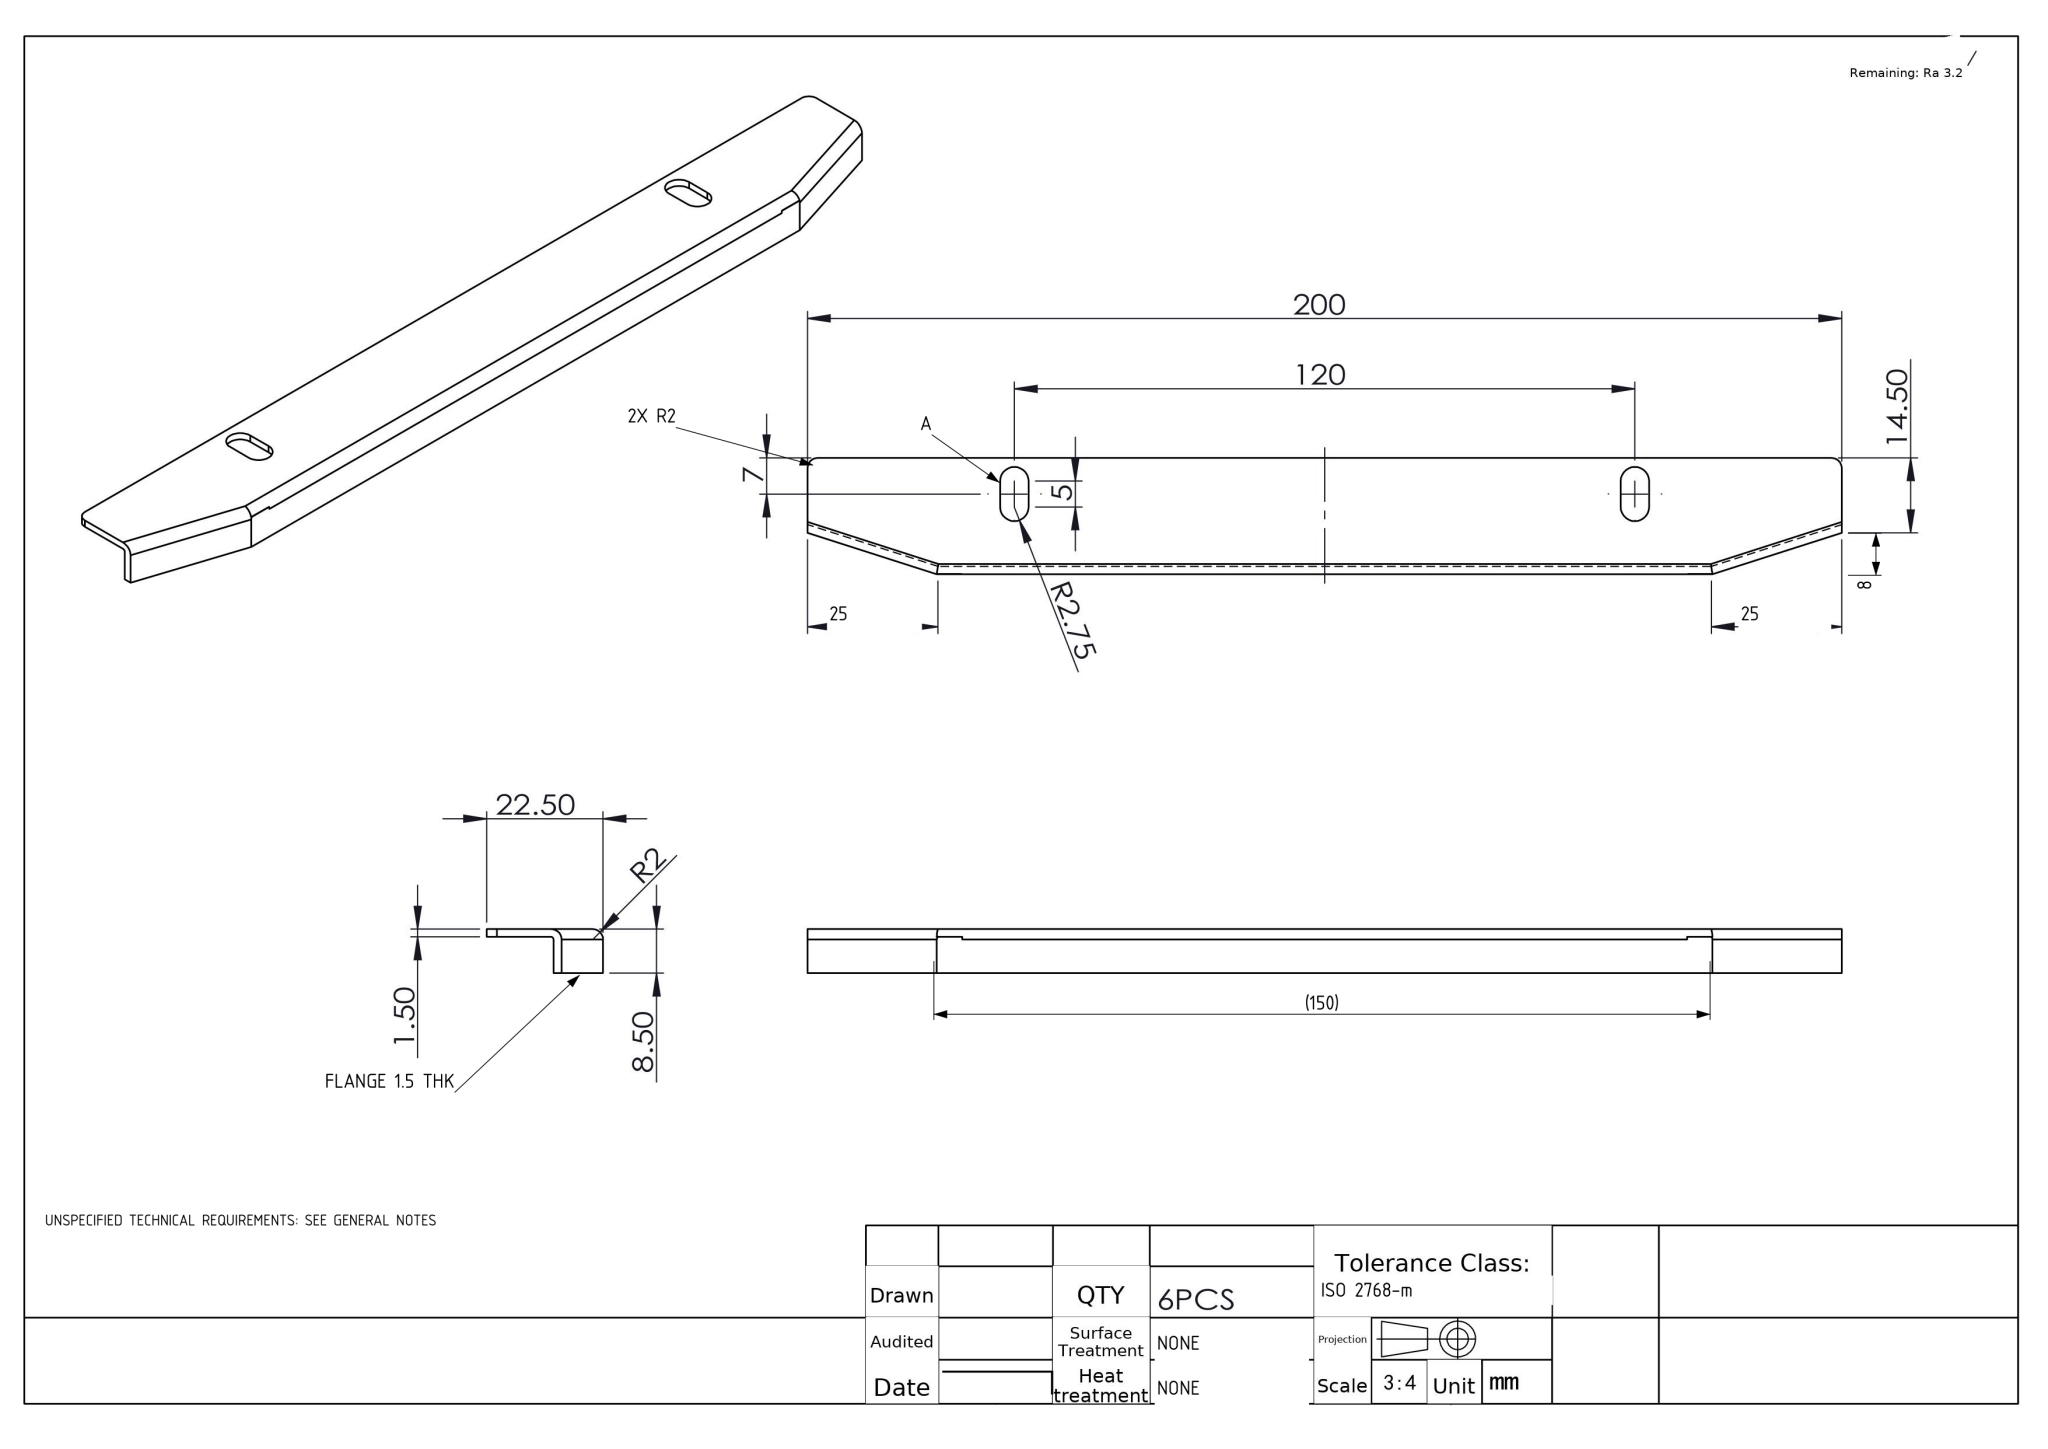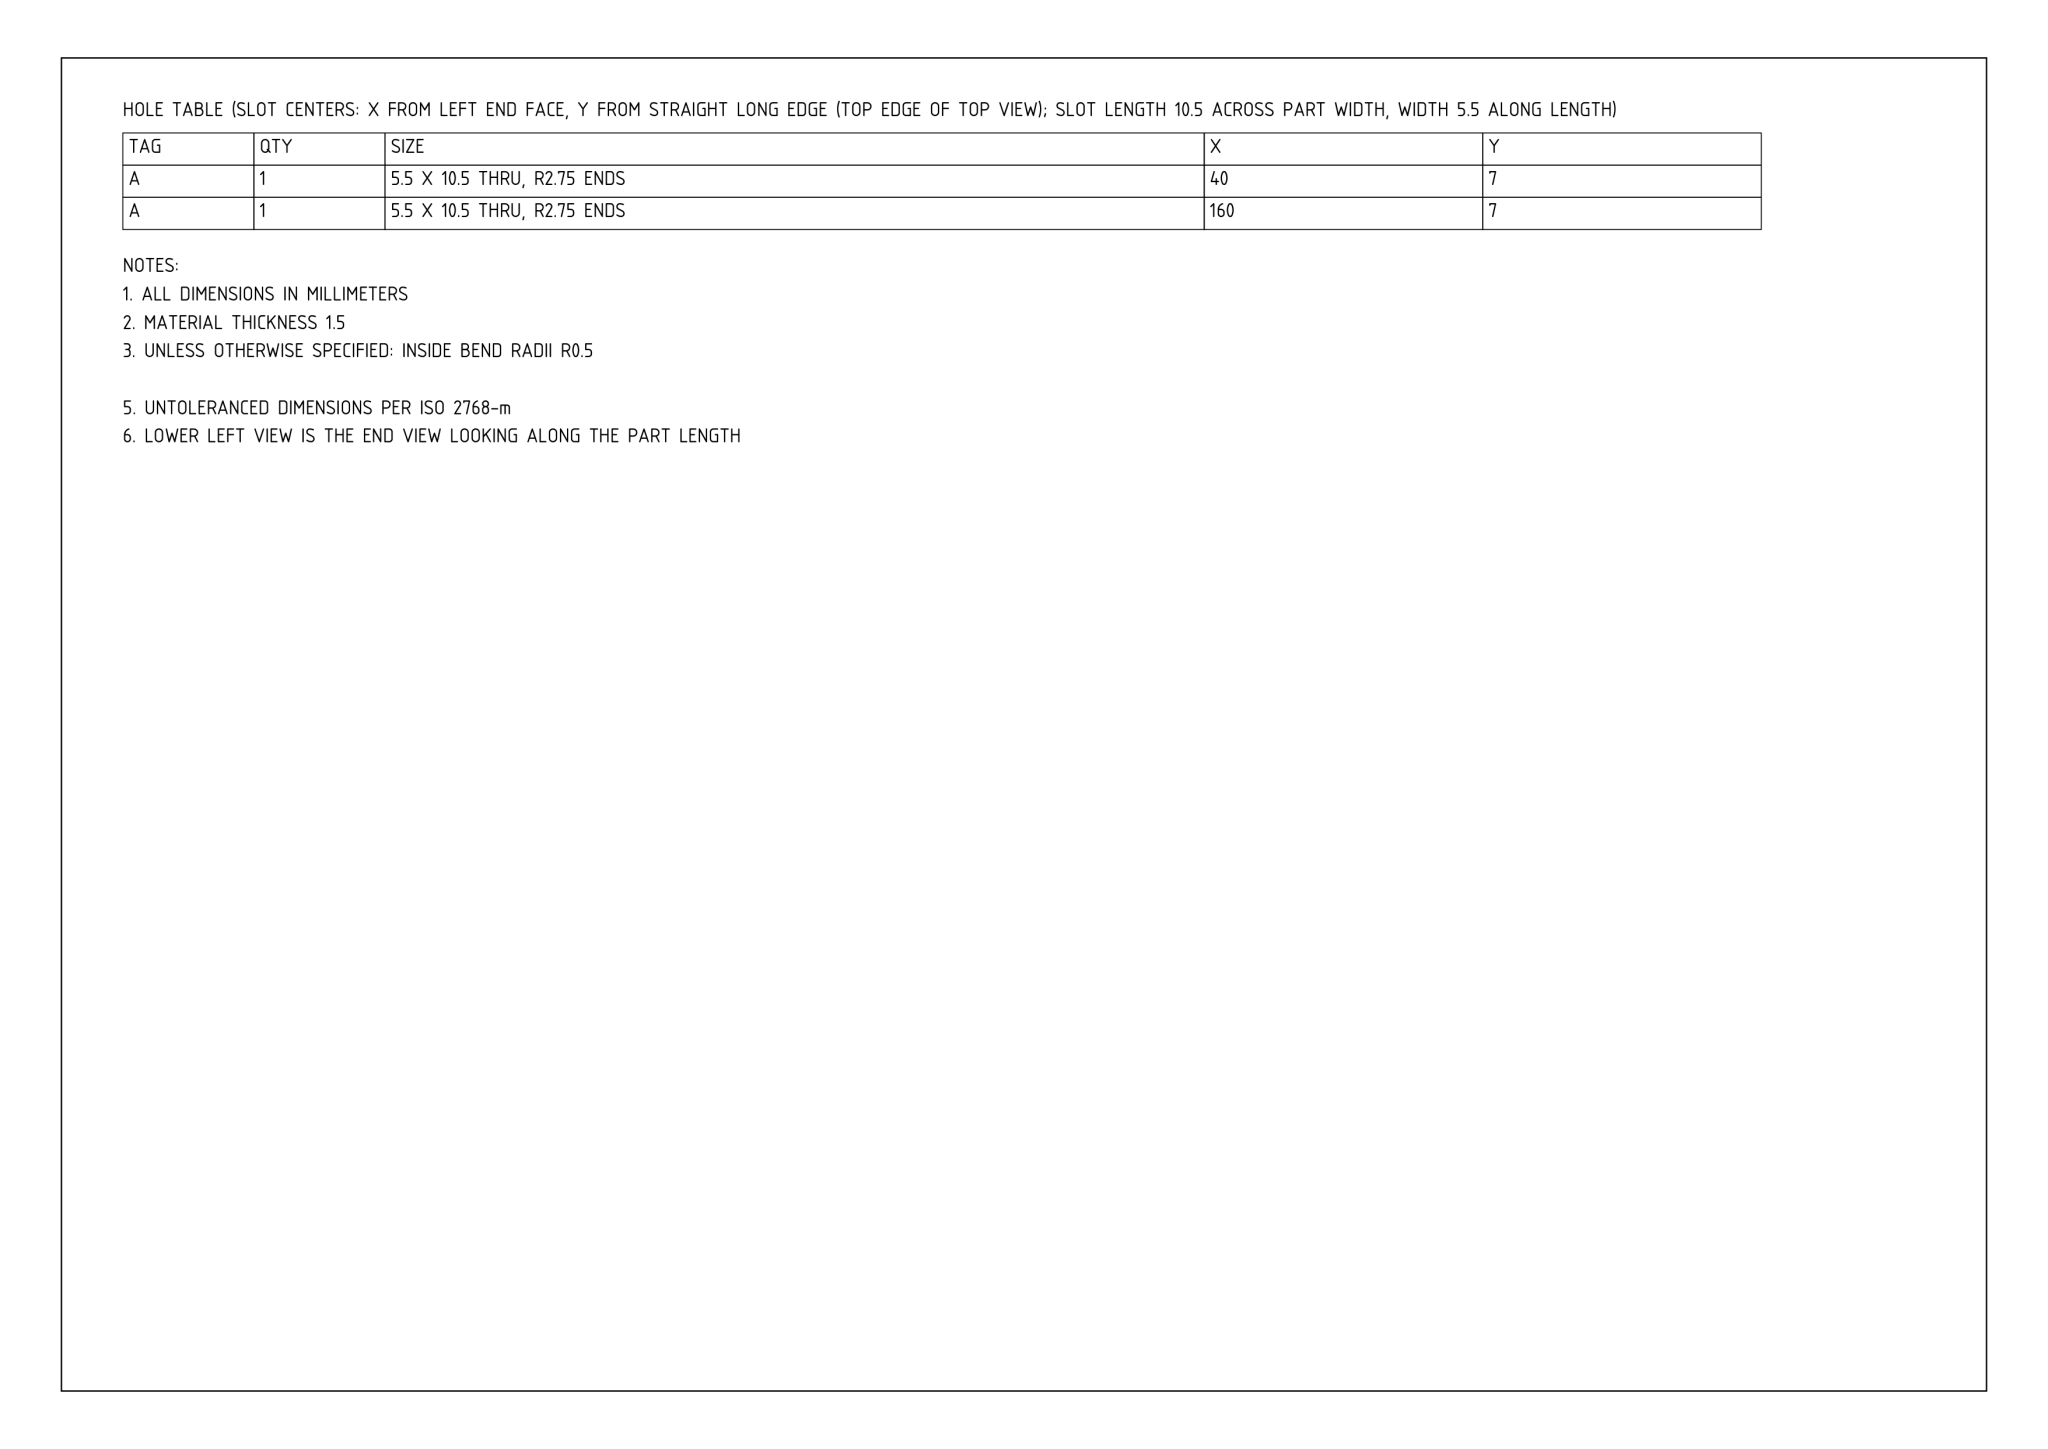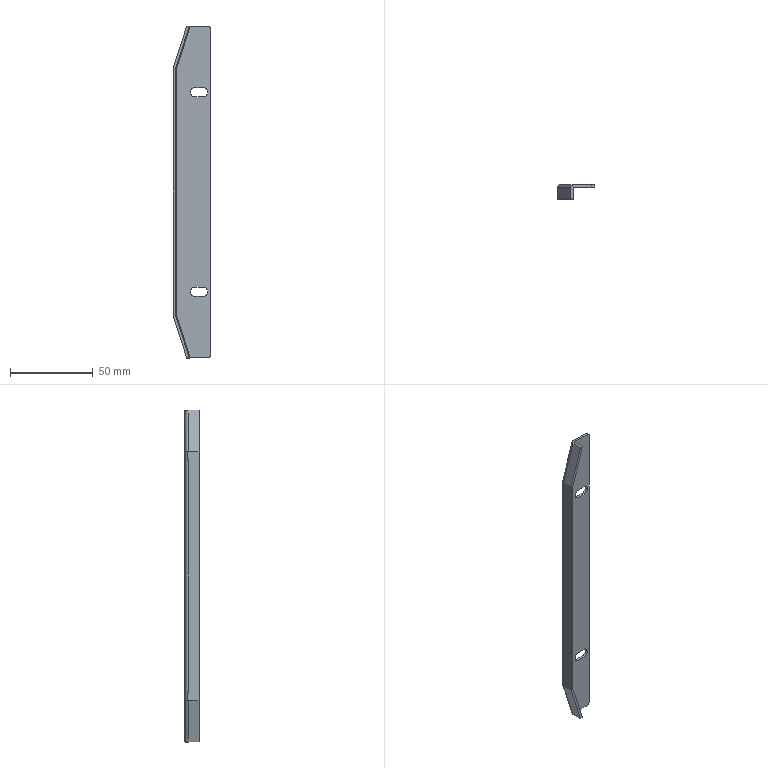Part | NX | mm | 1 solid | 36 faces | box 22.5 x 8.5 x 200 mm | volume 8257 mm3 | plane 20 | cylinder 14 | sphere 2 | commonest cylinder face diameters 1 x5 4 x5 5.5 x4